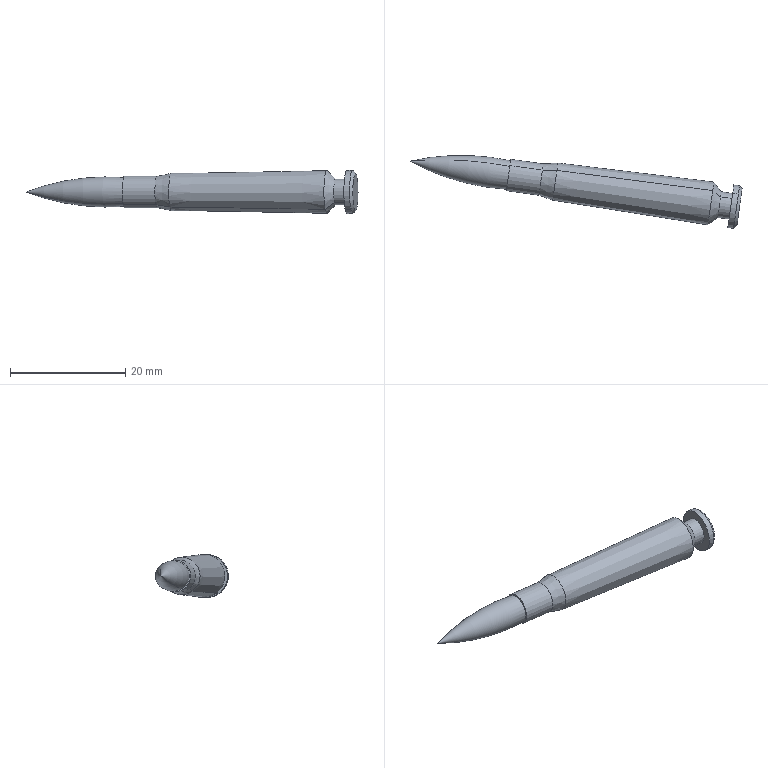Component | SolidWorks | Bullet-1 | 1 solid | 19 faces | box 57.69 x 12.69 x 7.5 mm | volume 1626 mm3 | cone 8 | cylinder 6 | plane 3 | torus 2 | commonest cylinder face diameters 7.5 x2 4.5 x2 5.5 x2
build123d program:
from build123d import *

# Parameters (mm, degrees)
CHAMFER1_SIZE = 0.5


with BuildPart() as part:
    # Sketch1 → Revolve2 (revolve)
    with BuildSketch(Plane.XY, mode=Mode.PRIVATE) as revolve2_sk:
        with BuildLine():
            Line((0, 0), (0, 3.75))
            Line((0, 3.75), (1.5, 3.75))
            Line((1.5, 3.75), (1.5, 2.25))
            Line((1.5, 2.25), (3.5, 2.25))
            Line((3.5, 2.25), (5, 3.75))
            Line((5, 3.75), (32.3, 3.25))
            Line((32.3, 3.25), (34.8, 2.75))
            Line((34.8, 2.75), (40.5, 2.75))
            Line((40.5, 2.75), (40.5, 2.5))
            ThreePointArc((40.5, 2.5), (49.288, 2.207), (57.8, 0))
            Line((57.8, 0), (0, 0))
        make_face()
    revolve(revolve2_sk.sketch.rotate(Axis((0, 0, 0), (1, 0, 0)), 90), axis=Axis((0, 0, 0), (1, 0, 0)))

    # Chamfer1
    chamfer1_edges = [part.edges().sort_by_distance(p)[0] for p in [
        (0, 0, -3.75),
    ]]
    chamfer(chamfer1_edges, length=CHAMFER1_SIZE)


solid = part.part

# Placed as in the assembly
solid = solid.moved(Location((-0.1726, -24.177, 1009.12), (-9.722, 1.359, 172.116)))
STEP:
#1=COLOUR_RGB('',0.7922,0.8196,0.9333);
#2=FILL_AREA_STYLE_COLOUR('',#1);
#3=FILL_AREA_STYLE('',(#2));
#4=SURFACE_STYLE_FILL_AREA(#3);
#5=SURFACE_SIDE_STYLE('',(#4));
#6=SURFACE_STYLE_USAGE(.BOTH.,#5);
#7=PRESENTATION_STYLE_ASSIGNMENT((#6));
#8=CARTESIAN_POINT('',(-0.01748,-1.028,39.627));
#9=VERTEX_POINT('',#8);
#10=CARTESIAN_POINT('',(0.003897,-0.8758,39.831));
#11=VERTEX_POINT('',#10);
#12=CARTESIAN_POINT('',(-0.006794,-0.9518,39.729));
#13=DIRECTION('',(0.9903,-0.1392,0.));
#14=DIRECTION('',(0.08355,0.5945,0.7997));
#15=AXIS2_PLACEMENT_3D('',#12,#13,#14);
#16=CIRCLE('',#15,0.128);
#17=EDGE_CURVE('',#9,#11,#16,.T.);
#18=ORIENTED_EDGE('',*,*,#17,.F.);
#19=CARTESIAN_POINT('',(-0.03862,-1.037,39.611));
#20=VERTEX_POINT('',#19);
#21=CARTESIAN_POINT('',(-0.01748,-1.028,39.627));
#22=DIRECTION('',(-0.7593,-0.322,-0.5655));
#23=VECTOR('',#22,39.37);
#24=LINE('',#21,#23);
#25=EDGE_CURVE('',#9,#20,#24,.T.);
#26=ORIENTED_EDGE('',*,*,#25,.T.);
#27=CARTESIAN_POINT('',(-0.01395,-0.8613,39.847));
#28=VERTEX_POINT('',#27);
#29=CARTESIAN_POINT('',(-0.02629,-0.9491,39.729));
#30=DIRECTION('',(-0.9903,0.1392,-0.));
#31=DIRECTION('',(0.08355,0.5945,0.7997));
#32=AXIS2_PLACEMENT_3D('',#29,#30,#31);
#33=CIRCLE('',#32,0.1476);
#34=EDGE_CURVE('',#28,#20,#33,.T.);
#35=ORIENTED_EDGE('',*,*,#34,.F.);
#36=CARTESIAN_POINT('',(0.003897,-0.8758,39.831));
#37=DIRECTION('',(-0.6411,0.5188,0.5655));
#38=VECTOR('',#37,39.37);
#39=LINE('',#36,#38);
#40=EDGE_CURVE('',#11,#28,#39,.T.);
#41=ORIENTED_EDGE('',*,*,#40,.F.);
#42=EDGE_LOOP('',(#18,#26,#35,#41));
#43=FACE_OUTER_BOUND('',#42,.T.);
#44=CARTESIAN_POINT('',(-0.006794,-0.9518,39.729));
#45=DIRECTION('',(-0.9903,0.1392,-0.));
#46=DIRECTION('',(0.08355,0.5945,0.7997));
#47=AXIS2_PLACEMENT_3D('',#44,#45,#46);
#48=CONICAL_SURFACE('',#47,0.128,0.7854);
#49=ADVANCED_FACE('',(#43),#48,.T.);
#50=CARTESIAN_POINT('',(-2.26,-0.6351,39.729));
#51=VERTEX_POINT('',#50);
#52=CARTESIAN_POINT('',(-1.594,-0.7885,39.65));
#53=VERTEX_POINT('',#52);
#54=CARTESIAN_POINT('',(-1.582,0.1618,40.906));
#55=DIRECTION('',(-0.1113,-0.792,0.6003));
#56=DIRECTION('',(0.,-0.6041,-0.7969));
#57=AXIS2_PLACEMENT_3D('',#54,#55,#56);
#58=CIRCLE('',#57,1.575);
#59=EDGE_CURVE('',#51,#53,#58,.T.);
#60=ORIENTED_EDGE('',*,*,#59,.F.);
#61=CARTESIAN_POINT('',(-1.578,-0.6714,39.808));
#62=VERTEX_POINT('',#61);
#63=CARTESIAN_POINT('',(-1.828,-1.588,38.552));
#64=DIRECTION('',(0.1113,0.792,-0.6003));
#65=DIRECTION('',(0.,0.6041,0.7969));
#66=AXIS2_PLACEMENT_3D('',#63,#64,#65);
#67=CIRCLE('',#66,1.575);
#68=EDGE_CURVE('',#51,#62,#67,.T.);
#69=ORIENTED_EDGE('',*,*,#68,.T.);
#70=CARTESIAN_POINT('',(-1.586,-0.7299,39.729));
#71=DIRECTION('',(0.9903,-0.1392,0.));
#72=DIRECTION('',(-0.08355,-0.5945,-0.7997));
#73=AXIS2_PLACEMENT_3D('',#70,#71,#72);
#74=CIRCLE('',#73,0.09843);
#75=EDGE_CURVE('',#53,#62,#74,.T.);
#76=ORIENTED_EDGE('',*,*,#75,.F.);
#77=EDGE_LOOP('',(#60,#69,#76));
#78=FACE_OUTER_BOUND('',#77,.T.);
#79=CARTESIAN_POINT('',(-1.705,-0.7131,39.729));
#80=DIRECTION('',(0.9903,-0.1392,0.));
#81=DIRECTION('',(-0.08355,-0.5945,-0.7997));
#82=AXIS2_PLACEMENT_3D('',#79,#80,#81);
#83=TOROIDAL_SURFACE('',#82,-1.472,1.575);
#84=ADVANCED_FACE('',(#78),#83,.T.);
#85=CARTESIAN_POINT('',(-1.595,-0.7943,39.643));
#86=VERTEX_POINT('',#85);
#87=CARTESIAN_POINT('',(-1.577,-0.6656,39.816));
#88=VERTEX_POINT('',#87);
#89=CARTESIAN_POINT('',(-1.586,-0.7299,39.729));
#90=DIRECTION('',(0.9903,-0.1392,0.));
#91=DIRECTION('',(-0.08355,-0.5945,-0.7997));
#92=AXIS2_PLACEMENT_3D('',#89,#90,#91);
#93=CIRCLE('',#92,0.1083);
#94=EDGE_CURVE('',#86,#88,#93,.T.);
#95=ORIENTED_EDGE('',*,*,#94,.T.);
#96=CARTESIAN_POINT('',(-1.354,-0.6968,39.816));
#97=VERTEX_POINT('',#96);
#98=CARTESIAN_POINT('',(0.002252,-0.8875,39.816));
#99=DIRECTION('',(0.9903,-0.1392,0.));
#100=VECTOR('',#99,39.37);
#101=LINE('',#98,#100);
#102=EDGE_CURVE('',#88,#97,#101,.T.);
#103=ORIENTED_EDGE('',*,*,#102,.T.);
#104=CARTESIAN_POINT('',(-1.373,-0.8255,39.643));
#105=VERTEX_POINT('',#104);
#106=CARTESIAN_POINT('',(-1.364,-0.7612,39.729));
#107=DIRECTION('',(0.9903,-0.1392,0.));
#108=DIRECTION('',(-0.08355,-0.5945,-0.7997));
#109=AXIS2_PLACEMENT_3D('',#106,#107,#108);
#110=CIRCLE('',#109,0.1083);
#111=EDGE_CURVE('',#105,#97,#110,.T.);
#112=ORIENTED_EDGE('',*,*,#111,.F.);
#113=CARTESIAN_POINT('',(-0.01584,-1.016,39.643));
#114=DIRECTION('',(0.9903,-0.1392,0.));
#115=VECTOR('',#114,39.37);
#116=LINE('',#113,#115);
#117=EDGE_CURVE('',#86,#105,#116,.T.);
#118=ORIENTED_EDGE('',*,*,#117,.F.);
#119=EDGE_LOOP('',(#95,#103,#112,#118));
#120=FACE_OUTER_BOUND('',#119,.T.);
#121=CARTESIAN_POINT('',(-0.006794,-0.9518,39.729));
#122=DIRECTION('',(0.9903,-0.1392,0.));
#123=DIRECTION('',(-0.08355,-0.5945,-0.7997));
#124=AXIS2_PLACEMENT_3D('',#121,#122,#123);
#125=CYLINDRICAL_SURFACE('',#124,0.1083);
#126=ADVANCED_FACE('',(#120),#125,.T.);
#127=ORIENTED_EDGE('',*,*,#111,.T.);
#128=CARTESIAN_POINT('',(-1.255,-0.6988,39.831));
#129=VERTEX_POINT('',#128);
#130=CARTESIAN_POINT('',(-1.354,-0.6968,39.816));
#131=DIRECTION('',(0.9874,-0.01988,0.1568));
#132=VECTOR('',#131,39.37);
#133=LINE('',#130,#132);
#134=EDGE_CURVE('',#97,#129,#133,.T.);
#135=ORIENTED_EDGE('',*,*,#134,.T.);
#136=CARTESIAN_POINT('',(-1.277,-0.8509,39.627));
#137=VERTEX_POINT('',#136);
#138=CARTESIAN_POINT('',(-1.266,-0.7749,39.729));
#139=DIRECTION('',(0.9903,-0.1392,0.));
#140=DIRECTION('',(-0.08355,-0.5945,-0.7997));
#141=AXIS2_PLACEMENT_3D('',#138,#139,#140);
#142=CIRCLE('',#141,0.128);
#143=EDGE_CURVE('',#137,#129,#142,.T.);
#144=ORIENTED_EDGE('',*,*,#143,.F.);
#145=CARTESIAN_POINT('',(-1.373,-0.8255,39.643));
#146=DIRECTION('',(0.9547,-0.2531,-0.1568));
#147=VECTOR('',#146,39.37);
#148=LINE('',#145,#147);
#149=EDGE_CURVE('',#105,#137,#148,.T.);
#150=ORIENTED_EDGE('',*,*,#149,.F.);
#151=EDGE_LOOP('',(#127,#135,#144,#150));
#152=FACE_OUTER_BOUND('',#151,.T.);
#153=CARTESIAN_POINT('',(-1.364,-0.7612,39.729));
#154=DIRECTION('',(0.9903,-0.1392,0.));
#155=DIRECTION('',(-0.08355,-0.5945,-0.7997));
#156=AXIS2_PLACEMENT_3D('',#153,#154,#155);
#157=CONICAL_SURFACE('',#156,0.1083,0.1974);
#158=ADVANCED_FACE('',(#152),#157,.T.);
#159=ORIENTED_EDGE('',*,*,#143,.T.);
#160=CARTESIAN_POINT('',(-0.1894,-0.8367,39.847));
#161=VERTEX_POINT('',#160);
#162=CARTESIAN_POINT('',(-1.255,-0.6988,39.831));
#163=DIRECTION('',(0.9916,-0.1283,0.01464));
#164=VECTOR('',#163,39.37);
#165=LINE('',#162,#164);
#166=EDGE_CURVE('',#129,#161,#165,.T.);
#167=ORIENTED_EDGE('',*,*,#166,.T.);
#168=CARTESIAN_POINT('',(-0.2141,-1.012,39.611));
#169=VERTEX_POINT('',#168);
#170=CARTESIAN_POINT('',(-0.2017,-0.9245,39.729));
#171=DIRECTION('',(0.9903,-0.1392,0.));
#172=DIRECTION('',(-0.08355,-0.5945,-0.7997));
#173=AXIS2_PLACEMENT_3D('',#170,#171,#172);
#174=CIRCLE('',#173,0.1476);
#175=EDGE_CURVE('',#169,#161,#174,.T.);
#176=ORIENTED_EDGE('',*,*,#175,.F.);
#177=CARTESIAN_POINT('',(-1.277,-0.8509,39.627));
#178=DIRECTION('',(0.9886,-0.15,-0.01464));
#179=VECTOR('',#178,39.37);
#180=LINE('',#177,#179);
#181=EDGE_CURVE('',#137,#169,#180,.T.);
#182=ORIENTED_EDGE('',*,*,#181,.F.);
#183=EDGE_LOOP('',(#159,#167,#176,#182));
#184=FACE_OUTER_BOUND('',#183,.T.);
#185=CARTESIAN_POINT('',(-1.266,-0.7749,39.729));
#186=DIRECTION('',(0.9903,-0.1392,0.));
#187=DIRECTION('',(-0.08355,-0.5945,-0.7997));
#188=AXIS2_PLACEMENT_3D('',#185,#186,#187);
#189=CONICAL_SURFACE('',#188,0.128,0.01831);
#190=ADVANCED_FACE('',(#184),#189,.T.);
#191=CARTESIAN_POINT('',(-0.1506,-0.9853,39.658));
#192=VERTEX_POINT('',#191);
#193=CARTESIAN_POINT('',(-0.1358,-0.88,39.8));
#194=VERTEX_POINT('',#193);
#195=CARTESIAN_POINT('',(-0.1432,-0.9327,39.729));
#196=DIRECTION('',(0.9903,-0.1392,0.));
#197=DIRECTION('',(-0.08355,-0.5945,-0.7997));
#198=AXIS2_PLACEMENT_3D('',#195,#196,#197);
#199=CIRCLE('',#198,0.08858);
#200=EDGE_CURVE('',#192,#194,#199,.T.);
#201=ORIENTED_EDGE('',*,*,#200,.F.);
#202=CARTESIAN_POINT('',(-0.2141,-1.012,39.611));
#203=DIRECTION('',(-0.7593,-0.322,-0.5655));
#204=VECTOR('',#203,39.37);
#205=LINE('',#202,#204);
#206=EDGE_CURVE('',#192,#169,#205,.T.);
#207=ORIENTED_EDGE('',*,*,#206,.T.);
#208=ORIENTED_EDGE('',*,*,#175,.T.);
#209=CARTESIAN_POINT('',(-0.1894,-0.8367,39.847));
#210=DIRECTION('',(-0.6411,0.5188,0.5655));
#211=VECTOR('',#210,39.37);
#212=LINE('',#209,#211);
#213=EDGE_CURVE('',#194,#161,#212,.T.);
#214=ORIENTED_EDGE('',*,*,#213,.F.);
#215=EDGE_LOOP('',(#201,#207,#208,#214));
#216=FACE_OUTER_BOUND('',#215,.T.);
#217=CARTESIAN_POINT('',(-0.2017,-0.9245,39.729));
#218=DIRECTION('',(-0.9903,0.1392,-0.));
#219=DIRECTION('',(0.08355,0.5945,0.7997));
#220=AXIS2_PLACEMENT_3D('',#217,#218,#219);
#221=CONICAL_SURFACE('',#220,0.1476,0.7854);
#222=ADVANCED_FACE('',(#216),#221,.T.);
#223=ORIENTED_EDGE('',*,*,#200,.T.);
#224=CARTESIAN_POINT('',(-0.05787,-0.891,39.8));
#225=VERTEX_POINT('',#224);
#226=CARTESIAN_POINT('',(0.0006073,-0.8992,39.8));
#227=DIRECTION('',(0.9903,-0.1392,0.));
#228=VECTOR('',#227,39.37);
#229=LINE('',#226,#228);
#230=EDGE_CURVE('',#194,#225,#229,.T.);
#231=ORIENTED_EDGE('',*,*,#230,.T.);
#232=CARTESIAN_POINT('',(-0.07268,-0.9963,39.658));
#233=VERTEX_POINT('',#232);
#234=CARTESIAN_POINT('',(-0.06527,-0.9436,39.729));
#235=DIRECTION('',(0.9903,-0.1392,0.));
#236=DIRECTION('',(-0.08355,-0.5945,-0.7997));
#237=AXIS2_PLACEMENT_3D('',#234,#235,#236);
#238=CIRCLE('',#237,0.08858);
#239=EDGE_CURVE('',#233,#225,#238,.T.);
#240=ORIENTED_EDGE('',*,*,#239,.F.);
#241=CARTESIAN_POINT('',(-0.0142,-1.005,39.658));
#242=DIRECTION('',(0.9903,-0.1392,0.));
#243=VECTOR('',#242,39.37);
#244=LINE('',#241,#243);
#245=EDGE_CURVE('',#192,#233,#244,.T.);
#246=ORIENTED_EDGE('',*,*,#245,.F.);
#247=EDGE_LOOP('',(#223,#231,#240,#246));
#248=FACE_OUTER_BOUND('',#247,.T.);
#249=CARTESIAN_POINT('',(-0.006794,-0.9518,39.729));
#250=DIRECTION('',(0.9903,-0.1392,0.));
#251=DIRECTION('',(-0.08355,-0.5945,-0.7997));
#252=AXIS2_PLACEMENT_3D('',#249,#250,#251);
#253=CYLINDRICAL_SURFACE('',#252,0.08858);
#254=ADVANCED_FACE('',(#248),#253,.T.);
#255=CARTESIAN_POINT('',(-0.07761,-1.031,39.611));
#256=VERTEX_POINT('',#255);
#257=CARTESIAN_POINT('',(-0.05294,-0.8559,39.847));
#258=VERTEX_POINT('',#257);
#259=CARTESIAN_POINT('',(-0.06527,-0.9436,39.729));
#260=DIRECTION('',(0.9903,-0.1392,0.));
#261=DIRECTION('',(-0.08355,-0.5945,-0.7997));
#262=AXIS2_PLACEMENT_3D('',#259,#260,#261);
#263=CIRCLE('',#262,0.1476);
#264=EDGE_CURVE('',#256,#258,#263,.T.);
#265=ORIENTED_EDGE('',*,*,#264,.T.);
#266=CARTESIAN_POINT('',(0.005542,-0.8641,39.847));
#267=DIRECTION('',(0.9903,-0.1392,0.));
#268=VECTOR('',#267,39.37);
#269=LINE('',#266,#268);
#270=EDGE_CURVE('',#258,#28,#269,.T.);
#271=ORIENTED_EDGE('',*,*,#270,.T.);
#272=ORIENTED_EDGE('',*,*,#34,.T.);
#273=CARTESIAN_POINT('',(-0.01913,-1.04,39.611));
#274=DIRECTION('',(0.9903,-0.1392,0.));
#275=VECTOR('',#274,39.37);
#276=LINE('',#273,#275);
#277=EDGE_CURVE('',#256,#20,#276,.T.);
#278=ORIENTED_EDGE('',*,*,#277,.F.);
#279=EDGE_LOOP('',(#265,#271,#272,#278));
#280=FACE_OUTER_BOUND('',#279,.T.);
#281=CARTESIAN_POINT('',(-0.006794,-0.9518,39.729));
#282=DIRECTION('',(0.9903,-0.1392,0.));
#283=DIRECTION('',(-0.08355,-0.5945,-0.7997));
#284=AXIS2_PLACEMENT_3D('',#281,#282,#283);
#285=CYLINDRICAL_SURFACE('',#284,0.1476);
#286=ADVANCED_FACE('',(#280),#285,.T.);
#287=CARTESIAN_POINT('',(-0.006794,-0.9518,39.729));
#288=DIRECTION('',(0.9903,-0.1392,0.));
#289=DIRECTION('',(0.08355,0.5945,0.7997));
#290=AXIS2_PLACEMENT_3D('',#287,#288,#289);
#291=CIRCLE('',#290,0.128);
#292=EDGE_CURVE('',#11,#9,#291,.T.);
#293=ORIENTED_EDGE('',*,*,#292,.T.);
#294=ORIENTED_EDGE('',*,*,#17,.T.);
#295=EDGE_LOOP('',(#293,#294));
#296=FACE_OUTER_BOUND('',#295,.T.);
#297=CARTESIAN_POINT('',(-0.006794,-0.9518,39.729));
#298=DIRECTION('',(-0.9903,0.1392,-0.));
#299=DIRECTION('',(0.08355,0.5945,0.7997));
#300=AXIS2_PLACEMENT_3D('',#297,#298,#299);
#301=PLANE('',#300);
#302=ADVANCED_FACE('',(#296),#301,.F.);
#303=ORIENTED_EDGE('',*,*,#270,.F.);
#304=CARTESIAN_POINT('',(-0.06527,-0.9436,39.729));
#305=DIRECTION('',(0.9903,-0.1392,0.));
#306=DIRECTION('',(-0.08355,-0.5945,-0.7997));
#307=AXIS2_PLACEMENT_3D('',#304,#305,#306);
#308=CIRCLE('',#307,0.1476);
#309=EDGE_CURVE('',#258,#256,#308,.T.);
#310=ORIENTED_EDGE('',*,*,#309,.T.);
#311=ORIENTED_EDGE('',*,*,#277,.T.);
#312=CARTESIAN_POINT('',(-0.02629,-0.9491,39.729));
#313=DIRECTION('',(-0.9903,0.1392,-0.));
#314=DIRECTION('',(0.08355,0.5945,0.7997));
#315=AXIS2_PLACEMENT_3D('',#312,#313,#314);
#316=CIRCLE('',#315,0.1476);
#317=EDGE_CURVE('',#20,#28,#316,.T.);
#318=ORIENTED_EDGE('',*,*,#317,.T.);
#319=EDGE_LOOP('',(#303,#310,#311,#318));
#320=FACE_OUTER_BOUND('',#319,.T.);
#321=CARTESIAN_POINT('',(-0.006794,-0.9518,39.729));
#322=DIRECTION('',(0.9903,-0.1392,0.));
#323=DIRECTION('',(-0.08355,-0.5945,-0.7997));
#324=AXIS2_PLACEMENT_3D('',#321,#322,#323);
#325=CYLINDRICAL_SURFACE('',#324,0.1476);
#326=ADVANCED_FACE('',(#320),#325,.T.);
#327=ORIENTED_EDGE('',*,*,#264,.F.);
#328=ORIENTED_EDGE('',*,*,#309,.F.);
#329=EDGE_LOOP('',(#327,#328));
#330=FACE_OUTER_BOUND('',#329,.T.);
#331=ORIENTED_EDGE('',*,*,#239,.T.);
#332=CARTESIAN_POINT('',(-0.06527,-0.9436,39.729));
#333=DIRECTION('',(0.9903,-0.1392,0.));
#334=DIRECTION('',(-0.08355,-0.5945,-0.7997));
#335=AXIS2_PLACEMENT_3D('',#332,#333,#334);
#336=CIRCLE('',#335,0.08858);
#337=EDGE_CURVE('',#225,#233,#336,.T.);
#338=ORIENTED_EDGE('',*,*,#337,.T.);
#339=EDGE_LOOP('',(#331,#338));
#340=FACE_BOUND('',#339,.T.);
#341=CARTESIAN_POINT('',(-0.05541,-0.8735,39.676));
#342=DIRECTION('',(0.9903,-0.1392,0.));
#343=DIRECTION('',(-0.08355,-0.5945,-0.7997));
#344=AXIS2_PLACEMENT_3D('',#341,#342,#343);
#345=PLANE('',#344);
#346=ADVANCED_FACE('',(#330,#340),#345,.F.);
#347=ORIENTED_EDGE('',*,*,#230,.F.);
#348=CARTESIAN_POINT('',(-0.1432,-0.9327,39.729));
#349=DIRECTION('',(0.9903,-0.1392,0.));
#350=DIRECTION('',(-0.08355,-0.5945,-0.7997));
#351=AXIS2_PLACEMENT_3D('',#348,#349,#350);
#352=CIRCLE('',#351,0.08858);
#353=EDGE_CURVE('',#194,#192,#352,.T.);
#354=ORIENTED_EDGE('',*,*,#353,.T.);
#355=ORIENTED_EDGE('',*,*,#245,.T.);
#356=ORIENTED_EDGE('',*,*,#337,.F.);
#357=EDGE_LOOP('',(#347,#354,#355,#356));
#358=FACE_OUTER_BOUND('',#357,.T.);
#359=CARTESIAN_POINT('',(-0.006794,-0.9518,39.729));
#360=DIRECTION('',(0.9903,-0.1392,0.));
#361=DIRECTION('',(-0.08355,-0.5945,-0.7997));
#362=AXIS2_PLACEMENT_3D('',#359,#360,#361);
#363=CYLINDRICAL_SURFACE('',#362,0.08858);
#364=ADVANCED_FACE('',(#358),#363,.T.);
#365=ORIENTED_EDGE('',*,*,#206,.F.);
#366=ORIENTED_EDGE('',*,*,#353,.F.);
#367=ORIENTED_EDGE('',*,*,#213,.T.);
#368=CARTESIAN_POINT('',(-0.2017,-0.9245,39.729));
#369=DIRECTION('',(0.9903,-0.1392,0.));
#370=DIRECTION('',(-0.08355,-0.5945,-0.7997));
#371=AXIS2_PLACEMENT_3D('',#368,#369,#370);
#372=CIRCLE('',#371,0.1476);
#373=EDGE_CURVE('',#161,#169,#372,.T.);
#374=ORIENTED_EDGE('',*,*,#373,.T.);
#375=EDGE_LOOP('',(#365,#366,#367,#374));
#376=FACE_OUTER_BOUND('',#375,.T.);
#377=CARTESIAN_POINT('',(-0.2017,-0.9245,39.729));
#378=DIRECTION('',(-0.9903,0.1392,-0.));
#379=DIRECTION('',(0.08355,0.5945,0.7997));
#380=AXIS2_PLACEMENT_3D('',#377,#378,#379);
#381=CONICAL_SURFACE('',#380,0.1476,0.7854);
#382=ADVANCED_FACE('',(#376),#381,.T.);
#383=ORIENTED_EDGE('',*,*,#166,.F.);
#384=CARTESIAN_POINT('',(-1.266,-0.7749,39.729));
#385=DIRECTION('',(0.9903,-0.1392,0.));
#386=DIRECTION('',(-0.08355,-0.5945,-0.7997));
#387=AXIS2_PLACEMENT_3D('',#384,#385,#386);
#388=CIRCLE('',#387,0.128);
#389=EDGE_CURVE('',#129,#137,#388,.T.);
#390=ORIENTED_EDGE('',*,*,#389,.T.);
#391=ORIENTED_EDGE('',*,*,#181,.T.);
#392=ORIENTED_EDGE('',*,*,#373,.F.);
#393=EDGE_LOOP('',(#383,#390,#391,#392));
#394=FACE_OUTER_BOUND('',#393,.T.);
#395=CARTESIAN_POINT('',(-1.266,-0.7749,39.729));
#396=DIRECTION('',(0.9903,-0.1392,0.));
#397=DIRECTION('',(-0.08355,-0.5945,-0.7997));
#398=AXIS2_PLACEMENT_3D('',#395,#396,#397);
#399=CONICAL_SURFACE('',#398,0.128,0.01831);
#400=ADVANCED_FACE('',(#394),#399,.T.);
#401=ORIENTED_EDGE('',*,*,#134,.F.);
#402=CARTESIAN_POINT('',(-1.364,-0.7612,39.729));
#403=DIRECTION('',(0.9903,-0.1392,0.));
#404=DIRECTION('',(-0.08355,-0.5945,-0.7997));
#405=AXIS2_PLACEMENT_3D('',#402,#403,#404);
#406=CIRCLE('',#405,0.1083);
#407=EDGE_CURVE('',#97,#105,#406,.T.);
#408=ORIENTED_EDGE('',*,*,#407,.T.);
#409=ORIENTED_EDGE('',*,*,#149,.T.);
#410=ORIENTED_EDGE('',*,*,#389,.F.);
#411=EDGE_LOOP('',(#401,#408,#409,#410));
#412=FACE_OUTER_BOUND('',#411,.T.);
#413=CARTESIAN_POINT('',(-1.364,-0.7612,39.729));
#414=DIRECTION('',(0.9903,-0.1392,0.));
#415=DIRECTION('',(-0.08355,-0.5945,-0.7997));
#416=AXIS2_PLACEMENT_3D('',#413,#414,#415);
#417=CONICAL_SURFACE('',#416,0.1083,0.1974);
#418=ADVANCED_FACE('',(#412),#417,.T.);
#419=ORIENTED_EDGE('',*,*,#102,.F.);
#420=CARTESIAN_POINT('',(-1.586,-0.7299,39.729));
#421=DIRECTION('',(0.9903,-0.1392,0.));
#422=DIRECTION('',(-0.08355,-0.5945,-0.7997));
#423=AXIS2_PLACEMENT_3D('',#420,#421,#422);
#424=CIRCLE('',#423,0.1083);
#425=EDGE_CURVE('',#88,#86,#424,.T.);
#426=ORIENTED_EDGE('',*,*,#425,.T.);
#427=ORIENTED_EDGE('',*,*,#117,.T.);
#428=ORIENTED_EDGE('',*,*,#407,.F.);
#429=EDGE_LOOP('',(#419,#426,#427,#428));
#430=FACE_OUTER_BOUND('',#429,.T.);
#431=CARTESIAN_POINT('',(-0.006794,-0.9518,39.729));
#432=DIRECTION('',(0.9903,-0.1392,0.));
#433=DIRECTION('',(-0.08355,-0.5945,-0.7997));
#434=AXIS2_PLACEMENT_3D('',#431,#432,#433);
#435=CYLINDRICAL_SURFACE('',#434,0.1083);
#436=ADVANCED_FACE('',(#430),#435,.T.);
#437=ORIENTED_EDGE('',*,*,#94,.F.);
#438=ORIENTED_EDGE('',*,*,#425,.F.);
#439=EDGE_LOOP('',(#437,#438));
#440=FACE_OUTER_BOUND('',#439,.T.);
#441=ORIENTED_EDGE('',*,*,#75,.T.);
#442=CARTESIAN_POINT('',(-1.586,-0.7299,39.729));
#443=DIRECTION('',(0.9903,-0.1392,0.));
#444=DIRECTION('',(-0.08355,-0.5945,-0.7997));
#445=AXIS2_PLACEMENT_3D('',#442,#443,#444);
#446=CIRCLE('',#445,0.09843);
#447=EDGE_CURVE('',#62,#53,#446,.T.);
#448=ORIENTED_EDGE('',*,*,#447,.T.);
#449=EDGE_LOOP('',(#441,#448));
#450=FACE_BOUND('',#449,.T.);
#451=CARTESIAN_POINT('',(-1.574,-0.6442,39.664));
#452=DIRECTION('',(0.9903,-0.1392,0.));
#453=DIRECTION('',(-0.08355,-0.5945,-0.7997));
#454=AXIS2_PLACEMENT_3D('',#451,#452,#453);
#455=PLANE('',#454);
#456=ADVANCED_FACE('',(#440,#450),#455,.F.);
#457=ORIENTED_EDGE('',*,*,#68,.F.);
#458=ORIENTED_EDGE('',*,*,#59,.T.);
#459=ORIENTED_EDGE('',*,*,#447,.F.);
#460=EDGE_LOOP('',(#457,#458,#459));
#461=FACE_OUTER_BOUND('',#460,.T.);
#462=CARTESIAN_POINT('',(-1.705,-0.7131,39.729));
#463=DIRECTION('',(0.9903,-0.1392,0.));
#464=DIRECTION('',(-0.08355,-0.5945,-0.7997));
#465=AXIS2_PLACEMENT_3D('',#462,#463,#464);
#466=TOROIDAL_SURFACE('',#465,-1.472,1.575);
#467=ADVANCED_FACE('',(#461),#466,.T.);
#468=ORIENTED_EDGE('',*,*,#25,.F.);
#469=ORIENTED_EDGE('',*,*,#292,.F.);
#470=ORIENTED_EDGE('',*,*,#40,.T.);
#471=ORIENTED_EDGE('',*,*,#317,.F.);
#472=EDGE_LOOP('',(#468,#469,#470,#471));
#473=FACE_OUTER_BOUND('',#472,.T.);
#474=CARTESIAN_POINT('',(-0.006794,-0.9518,39.729));
#475=DIRECTION('',(-0.9903,0.1392,-0.));
#476=DIRECTION('',(0.08355,0.5945,0.7997));
#477=AXIS2_PLACEMENT_3D('',#474,#475,#476);
#478=CONICAL_SURFACE('',#477,0.128,0.7854);
#479=ADVANCED_FACE('',(#473),#478,.T.);
#480=CLOSED_SHELL('',(#49,#84,#126,#158,#190,#222,#254,#286,#302,#326,#346,#364,#382,#400,#418,#436,#456,#467,#479));
#481=MANIFOLD_SOLID_BREP('',#480);
#482=STYLED_ITEM('',(#7),#481);
#483=PRESENTATION_LAYER_ASSIGNMENT('','',(#482));
#484=CARTESIAN_POINT('',(0.,0.,0.));
#485=DIRECTION('',(0.,0.,1.));
#486=DIRECTION('',(1.,0.,0.));
#487=AXIS2_PLACEMENT_3D('',#484,#485,#486);
#488=(LENGTH_UNIT()NAMED_UNIT(*)SI_UNIT($,.METRE.));
#489=LENGTH_MEASURE_WITH_UNIT(LENGTH_MEASURE(0.0254),#488);
#490=DIMENSIONAL_EXPONENTS(1.,0.,0.,0.,0.,0.,0.);
#491=(CONVERSION_BASED_UNIT('',#489)LENGTH_UNIT()NAMED_UNIT(#490));
#492=UNCERTAINTY_MEASURE_WITH_UNIT(LENGTH_MEASURE(0.00001),#491,'','');
#493=(NAMED_UNIT(*)PLANE_ANGLE_UNIT()SI_UNIT($,.RADIAN.));
#494=(NAMED_UNIT(*)SI_UNIT($,.STERADIAN.)SOLID_ANGLE_UNIT());
#495=(GEOMETRIC_REPRESENTATION_CONTEXT(3)GLOBAL_UNCERTAINTY_ASSIGNED_CONTEXT((#492))GLOBAL_UNIT_ASSIGNED_CONTEXT((#491,#493,#494))REPRESENTATION_CONTEXT('',''));
#496=ADVANCED_BREP_SHAPE_REPRESENTATION('',(#481,#487),#495);
#497=(LENGTH_UNIT()NAMED_UNIT(*)SI_UNIT($,.METRE.));
#498=LENGTH_MEASURE_WITH_UNIT(LENGTH_MEASURE(0.0254),#497);
#499=DIMENSIONAL_EXPONENTS(1.,0.,0.,0.,0.,0.,0.);
#500=(CONVERSION_BASED_UNIT('',#498)LENGTH_UNIT()NAMED_UNIT(#499));
#501=UNCERTAINTY_MEASURE_WITH_UNIT(LENGTH_MEASURE(0.00001),#500,'','');
#502=(NAMED_UNIT(*)PLANE_ANGLE_UNIT()SI_UNIT($,.RADIAN.));
#503=(NAMED_UNIT(*)SI_UNIT($,.STERADIAN.)SOLID_ANGLE_UNIT());
#504=(GEOMETRIC_REPRESENTATION_CONTEXT(3)GLOBAL_UNCERTAINTY_ASSIGNED_CONTEXT((#501))GLOBAL_UNIT_ASSIGNED_CONTEXT((#500,#502,#503))REPRESENTATION_CONTEXT('',''));
#505=MECHANICAL_DESIGN_GEOMETRIC_PRESENTATION_REPRESENTATION('',(#482),#504);